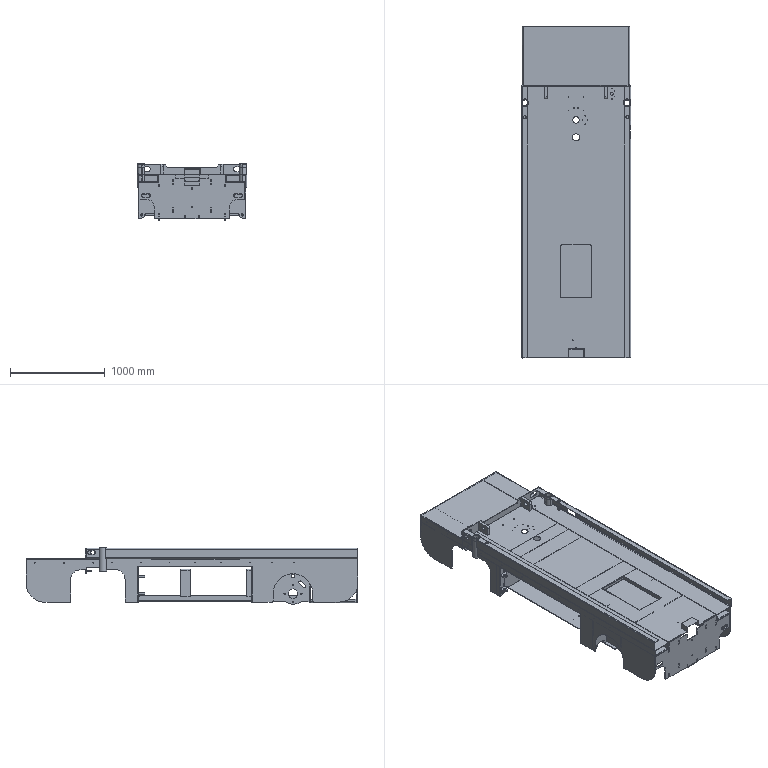Assembly | SolidWorks | mm | 35 component files | 35 solids | 1485 faces | box 1159 x 3506 x 598.09 mm | volume 81128529 mm3 | plane 1002 | cylinder 456 | cone 16 | spline 11 | commonest cylinder face diameters 7.2 x48 10 x40 20 x27 5.2 x24 8 x18 40 x17 30 x16 13.1 x16
Bill of materials:
BodyMainBoard | 1 | Q235 | Long rectangular plate formed from thin sheet, with a shallow flange bent up along each long edge (a shallow channel). It has a large rectangular cutout, several round holes near one end, and small tabs with holes at that end.
BodySidePlate,Right | 1 | Q235 | Long, narrow, thin profiled plate/bracket. One long edge is straight; the other has two downward legs and a large semicircular arch cutout between them. A narrow bent lip runs along part of the top edge.
BoxSupport,Left | 1 | Q235 | Long L-section angle formed from sheet, with one wide leg and one short upturned flange. The short flange has notches along its length, and one end has stepped notches.
BoxSupport,Right | 1 | Q235 | Long L-section angle formed from sheet, with notches along the short flange and a stepped notch profile at one end of the wide leg. It appears to be the opposite-hand version of a similar angle part.
BrakeMountingPlate | 2 | Q235 | Flat, roughly rectangular plate with small rectangular tabs on its side edges and a rounded lobe extending from the bottom edge. It has a large central round hole surrounded by four small holes, plus a separate round hole and a diagonal slot.
CounterweightFixingFrame | 2 | Q235 | U-shaped strap or bracket formed from thin sheet: a flat top web with two long parallel legs, and a single round hole in the center of the web.
ForkliftBasePlate | 2 | Q235 | Plain straight U-channel formed from sheet: a flat base with two parallel side walls of equal height and no visible holes.
ForkliftSidePlate,Left | 1 | Q235 | Long, slender L-section angle formed from sheet. It has a semicircular edge notch near one end, a hole in the upright flange, and several small slits or marks along the flat leg.
ForkliftSidePlate,Right | 1 | Q235 | Long, slender L-section angle, apparently the opposite-hand version of a similar part. It has a semicircular edge notch near one end, an obround hole in the flange, and small slits along the flat leg.
ForkLug | 2 | Q235 | Small, thick rectangular block or plate with one large rounded corner, one smaller rounded corner, and a single round through-hole.
FrontEndPlate,2 | 1 | Q235 | Flat, elongated thin plate with a straight top edge and a profiled bottom edge with chamfered steps. It has one centered obround slot near the bottom edge.
FrontEndPlate | 1 | Q235 | Flat, elongated thin plate with obround slots near both ends, a recessed or stepped profile along the top edge, and chamfered lower corners. Two small rectangular slots are near the center.
FrontGuard | 1 | Q235 | Thin-wall cover shaped like an inverted U: a flat rectangular top panel with two matching side panels bent down. Each side panel has a stepped tab at one end, a notch with a rounded inside corner, and a large-radius rounded corner at the other end.
FrontStiffener,Left | 1 | Q235 | Long thin L-shaped angle profile: a wide flat leg and a shorter upright leg joined by a rounded bend. One corner of the flat leg has a small chamfer.
FrontStiffener,Right | 1 | Q235 | Long thin L-shaped angle profile that looks like a mirror image of the similar angle part: a wide flat leg and an upright leg on the opposite side, joined by a rounded bend, with a small chamfer on one corner of the flat leg.
FrontUprightPlate | 1 | Q235 | Flat thin plate, roughly rectangular, with a raised centre section along the top edge, stepped edges, and many through-features: two vertical obround slots, several rectangular slots, small round holes, and rounded corner lugs with round holes at the two bottom corners.
LadderFixingPlate | 1 | Q235 | Flat thin plate with a stepped, castellated top edge and wide side wings. Each wing has a horizontal obround slot and a large-radius curved cut where it meets the narrower lower body. The plate has several narrow vertical rectangular slots and two small round holes on the centreline.
MainBoardLowerBucklePlate | 1 | Q235 | Shallow open rectangular tray: a flat rectangular base with short upright walls on all four sides.
ManualPumpProtectionBox | 1 | Q235 | Inverted U-shaped channel or cover: a flat rectangular top panel with two parallel side walls bent down at rounded bends, and small circular relief notches at the ends of the bends.
RearUprightPlate | 2 | Q235 | Flat thin plate, roughly rectangular, with a tall narrow tab rising at one upper corner, a small tab on the top edge, a rectangular slot near the top-left, two notches in the bottom edge, and a rounded lug with a round hole at the lower-right corner.
RearUprightPlateConnection | 1 | Q235 | Flat thin plate with a stepped top edge (two raised blocks with a recessed centre), wide side wings joined to a narrower lower body by large concave radii, narrow vertical rectangular slots near the corners, and small notches in the top and bottom edges. No obround slots or round holes are visible.
SteeringLug | 1 | Q235 | Small thick flat plate or bracket shaped roughly like a tapered trapezoid: one angled edge, a rectangular tab on the top edge, a rounded bottom end, and one large round through-hole near the rounded end.
Stiffener,RearConnection | 1 | Q235 | Long U-shaped channel: a flat base with two parallel upright side walls joined by rounded bends, with a constant cross-section along the length.
VehicleBodyLowerLug | 2 | Q235 | Small thick flat plate or bracket with a stepped top edge (two levels of rectangular steps), one straight side, an angled lower edge, a rounded bottom end, and one large round through-hole near the rounded end.
VehicleBodySidePlate,Left | 1 | Q235 | Long, thin, flat plate with a straight top edge. The left end has a large semicircular cutout open to the bottom edge and one rounded bottom corner. A long rectangular opening runs between two narrow vertical legs. Each leg has a short bent tab with small holes and a rounded end with a single larger hole. The right end has a concave radiused notch.
VehicleBodyUpperLug | 2 | Q235 | Flat plate of even thickness with a stepped, tapering outline. It has one round through-hole near a rounded lobe at one end. Opposite the hole, one edge is stepped like a staircase, and a long straight edge slants back toward the lobe.
VerticalShaftSleeve | 2 | Q235 | Straight hollow cylindrical tube with a thin wall and plain ends. It has one small radial hole through the wall, partway along its length.
Mates:
1. coincident | BodyMainBoard-1 face at (-1392.449, -1040.568, 2815.705) dir (0, 0, -1) | ForkliftSidePlate,Right-1 face at (-1178.654, 634.006, 2815.705) dir (0, 0, 1)
2. concentric | BodyMainBoard-1 face at (-1356.654, 1601.474, 2820.705) dir (0, 0, 1) r 40.25 | ForkliftSidePlate,Right-1 face at (-1356.654, 1601.474, 2740.705) dir (0, 0, 1) r 40.25
3. parallel | BodyMainBoard-1 face at (-1392.654, -1040.568, 2823.29) dir (-1, 0, 0) | ForkliftSidePlate,Right-1 face at (-1377.654, 634.006, 2740.705) dir (-1, 0, 0)
4. coincident | BodyMainBoard-1 face at (-1392.449, -1040.568, 2815.705) dir (0, 0, -1) | ForkliftSidePlate,Left-1 face at (-455.654, 634.006, 2815.705) dir (0, 0, 1)
5. concentric | BodyMainBoard-1 face at (-277.654, 1601.474, 2820.705) dir (0, 0, 1) r 40.25 | ForkliftSidePlate,Left-1 face at (-277.654, 1601.474, 2740.705) dir (0, 0, 1) r 40.25
6. coincident | ForkliftSidePlate,Right-1 face at (-1377.654, 634.006, 2740.705) dir (-1, 0, 0) | VehicleBodySidePlate,Left-1 face at (-1377.654, 1009.2, 2306.758) dir (1, 0, 0)
7. coincident | ForkliftSidePlate,Left-1 face at (-256.654, 634.006, 2740.705) dir (1, 0, 0) | BodySidePlate,Right-1 face at (-256.654, 1009.2, 2306.758) dir (-1, 0, 0)
8. coincident | BodyMainBoard-1 face at (-1392.449, -1040.568, 2815.705) dir (0, 0, -1) | BodySidePlate,Right-1 face at (-256.654, 1009.2, 2815.705) dir (0, 0, 1)
9. coincident | ForkliftSidePlate,Right-1 face at (-458.055, 634.006, 2735.705) dir (0, 0, -1) | FrontUprightPlate-1 face at (-2022.148, 1276.474, 2735.705) dir (0, 0, 1)
10. coincident | ForkliftSidePlate,Right-1 face at (-1343.154, 634.006, 2740.705) dir (1, 0, 0) | FrontUprightPlate-1 face at (-1343.154, 1276.474, 2221.675) dir (-1, 0, 0)
11. coincident | ForkliftSidePlate,Right-1 face at (-458.055, 1286.474, 2740.705) dir (0, -1, 0) | FrontUprightPlate-1 face at (-2022.148, 1286.474, 2221.675) dir (0, 1, 0)
12. coincident | ForkliftSidePlate,Left-1 face at (-1176.253, -155.326, 2740.705) dir (0, -1, 0) | RearUprightPlate-1 face at (3301.77, -155.326, 514.924) dir (0, 1, 0)
13. coincident | ForkliftSidePlate,Left-1 face at (-331.154, 634.006, 2740.705) dir (1, 0, 0) | RearUprightPlate-1 face at (-331.154, -155.326, 514.924) dir (-1, 0, 0)
14. coincident | ForkliftSidePlate,Right-1 face at (-458.055, -155.326, 2740.705) dir (0, -1, 0) | RearUprightPlate-2 face at (-4936.078, -155.326, 514.924) dir (0, 1, 0)
15. coincident | RearUprightPlate-1 face at (3301.77, -155.326, 2397.705) dir (0, 0, -1) | BrakeMountingPlate-1 face at (-470.054, -14.958, 2397.705) dir (0, 0, 1)
16. coincident | RearUprightPlate-1 face at (-460.054, -155.326, 514.924) dir (-1, 0, 0) | BrakeMountingPlate-1 face at (-460.054, -14.958, 2306.634) dir (1, 0, 0)
17. coincident | RearUprightPlate-1 face at (3301.77, -165.326, 514.924) dir (0, -1, 0) | BrakeMountingPlate-1 face at (-470.054, -165.326, 2306.634) dir (0, 1, 0)
18. coincident | RearUprightPlate-2 face at (-1174.254, -165.326, 514.924) dir (1, 0, 0) | BrakeMountingPlate-2 face at (-1174.254, -14.958, 2306.634) dir (-1, 0, 0)
19. coincident | RearUprightPlate-2 face at (-4936.078, -165.326, 514.924) dir (0, -1, 0) | BrakeMountingPlate-2 face at (-1174.254, -165.326, 2306.634) dir (0, 1, 0)
20. coincident | RearUprightPlate-2 face at (-4936.078, -165.326, 2397.705) dir (0, 0, -1) | BrakeMountingPlate-2 face at (-1174.254, -14.958, 2397.705) dir (0, 0, 1)
21. concentric | BodyMainBoard-1 face at (-1356.654, 1601.474, 2820.705) dir (0, 0, 1) r 40.25 | VerticalShaftSleeve-1 face at (-1356.654, 1601.474, 2678.295) dir (0, 0, 1) r 40
22. distance | VerticalShaftSleeve-1 face at (-1356.654, 1601.474, 2931.295) dir (0, 0, 1) | BodyMainBoard-1 face at (-1487.869, -1040.568, 2926.295) dir (0, 0, 1)
23. distance | VerticalShaftSleeve-2 face at (-277.654, 1601.474, 2931.295) dir (0, 0, 1) | BodyMainBoard-1 face at (1006.151, -1040.568, 2926.295) dir (0, 0, 1)
24. coincident | FrontUprightPlate-1 face at (-1307.654, 1276.474, 2221.675) dir (-1, 0, 0) | VehicleBodyLowerLug-1 face at (-1307.654, 1144.825, 2439.705) dir (1, 0, 0)
25. coincident | FrontUprightPlate-1 face at (-2022.148, 1276.474, 2439.705) dir (0, 0, 1) | VehicleBodyLowerLug-1 face at (-1381.214, 1144.825, 2439.705) dir (0, 0, -1)
26. coincident | FrontUprightPlate-1 face at (-2022.148, 1286.474, 2221.675) dir (0, 1, 0) | VehicleBodyLowerLug-1 face at (-1381.214, 1286.474, 2439.705) dir (0, 1, 0)
27. coincident | FrontUprightPlate-1 face at (-2022.148, 1276.474, 2439.721) dir (0, 0, 1) | VehicleBodyLowerLug-2 face at (-253.037, 1144.825, 2439.721) dir (0, 0, -1)
28. coincident | FrontUprightPlate-1 face at (-2022.148, 1286.474, 2221.675) dir (0, 1, 0) | VehicleBodyLowerLug-2 face at (-253.037, 1286.474, 2455.721) dir (0, 1, 0)
29. coincident | FrontUprightPlate-1 face at (-326.597, 1276.474, 2221.675) dir (1, 0, 0) | VehicleBodyLowerLug-2 edge at (-326.597, 1286.474, 2455.721) dir (0, 0, -1)
30. coincident | FrontUprightPlate-1 face at (-2022.148, 1276.474, 2619.521) dir (0, 0, 1) | VehicleBodyUpperLug-1 face at (-1424.9, 1092.251, 2619.521) dir (0, 0, -1)
31. coincident | FrontUprightPlate-1 face at (-2022.148, 1286.474, 2221.675) dir (0, 1, 0) | VehicleBodyUpperLug-1 face at (-1424.9, 1286.474, 2619.521) dir (0, 1, 0)
32. coincident | FrontUprightPlate-1 face at (-1257.654, 1276.474, 2221.675) dir (-1, 0, 0) | VehicleBodyUpperLug-1 face at (-1257.654, 1092.251, 2619.521) dir (1, 0, 0)
33. coincident | BrakeMountingPlate-1 face at (-470.054, -577.326, 2306.634) dir (0, -1, 0) | RearUprightPlateConnection-1 face at (-1412.879, -577.326, 2272.431) dir (0, 1, 0)
34. coincident | BrakeMountingPlate-1 face at (-470.054, -14.958, 2306.634) dir (-1, 0, 0) | RearUprightPlateConnection-1 face at (-470.054, -587.326, 2272.431) dir (1, 0, 0)
35. coincident | BodySidePlate,Right-1 face at (-475.431, 1226.474, 2306.758) dir (0, -1, 0) | VehicleBodyLowerLug-2 face at (-253.037, 1226.474, 2455.721) dir (0, 1, 0)
36. coincident | BodyMainBoard-1 face at (-1392.449, -1040.568, 2815.705) dir (0, 0, -1) | VehicleBodySidePlate,Left-1 face at (-1377.654, 1009.2, 2815.705) dir (0, 0, 1)
37. coincident | VehicleBodySidePlate,Left-1 face at (-1158.878, 1226.474, 2306.758) dir (0, -1, 0) | VehicleBodyUpperLug-1 face at (-1424.9, 1226.474, 2619.521) dir (0, 1, 0)
38. coincident | BodyMainBoard-1 face at (-1392.449, 1777.474, 2820.705) dir (0, 1, 0) | FrontEndPlate-1 face at (-1385.335, 1777.474, 2333.763) dir (0, -1, 0)
39. coincident | BodyMainBoard-1 face at (-240.654, -1040.568, 1671.7) dir (1, 0, 0) | FrontEndPlate-1 face at (-240.654, 1777.474, 2333.763) dir (1, 0, 0)
40. coincident | BodyMainBoard-1 face at (-1487.869, -1040.568, 2926.295) dir (0, 0, 1) | FrontEndPlate-1 face at (-1385.335, 1777.474, 2926.295) dir (0, 0, 1)
41. concentric | BodyMainBoard-1 face at (-277.654, 1601.474, 2820.705) dir (0, 0, 1) r 40.25 | VerticalShaftSleeve-2 face at (-277.654, 1601.474, 2678.295) dir (0, 0, 1) r 30.1
42. distance | FrontGuard-1 face at (-256.154, 1942.416, 4528.778) dir (-1, 0, 0) | ForkliftSidePlate,Left-1 face at (-256.654, 634.006, 2740.705) dir (1, 0, 0)
43. coincident | BodyMainBoard-1 face at (-1392.449, -1040.568, 2815.705) dir (0, 0, -1) | FrontGuard-1 face at (-1971.587, 1942.416, 2815.705) dir (0, 0, 1)
44. coincident | FrontEndPlate-1 face at (-1385.335, 1787.474, 2333.763) dir (0, 1, 0) | FrontGuard-1 face at (-1971.587, 1787.474, 2810.705) dir (0, -1, 0)
45. coincident | FrontGuard-1 face at (-1378.154, 1942.416, 2219.912) dir (1, 0, 0) | FrontStiffener,Left-1 face at (-1378.154, 2382.474, 2733.928) dir (-1, 0, 0)
46. coincident | FrontEndPlate-1 face at (-1385.335, 1787.474, 2333.763) dir (0, 1, 0) | FrontStiffener,Left-1 face at (-1176.514, 1787.474, 2806.289) dir (0, -1, 0)
47. coincident | FrontGuard-1 face at (-256.154, 1942.416, 4528.778) dir (-1, 0, 0) | FrontStiffener,Right-1 face at (-256.154, 2382.474, 2738.345) dir (1, 0, 0)
48. coincident | FrontGuard-1 face at (-1971.587, 1942.416, 2810.705) dir (0, 0, -1) | FrontStiffener,Right-1 face at (-457.794, 2402.474, 2810.705) dir (0, 0, 1)
49. coincident | FrontEndPlate-1 face at (-1385.335, 1787.474, 2333.763) dir (0, 1, 0) | FrontStiffener,Right-1 face at (-532.794, 1787.474, 2738.345) dir (0, -1, 0)
50. coincident | FrontStiffener,Right-1 face at (-532.794, 2402.474, 2738.345) dir (0, 1, 0) | FrontEndPlate,2-1 face at (-759.311, 2402.474, 2748.087) dir (0, -1, 0)
51. coincident | FrontGuard-1 face at (-256.154, 1942.416, 4528.778) dir (-1, 0, 0) | FrontEndPlate,2-1 face at (-256.154, 2412.474, 2748.087) dir (1, 0, 0)
52. coincident | FrontGuard-1 face at (-1971.587, 1942.416, 2810.705) dir (0, 0, -1) | FrontEndPlate,2-1 face at (-759.311, 2412.474, 2810.705) dir (0, 0, 1)
53. coincident | BodyMainBoard-1 face at (-1392.449, -1040.568, 2815.705) dir (0, 0, -1) | ForkliftBasePlate-1 face at (-460.654, 926.474, 2815.705) dir (0, 0, 1)
54. coincident | ForkliftSidePlate,Left-1 face at (-460.654, 634.006, 3459.094) dir (-1, 0, 0) | ForkliftBasePlate-1 face at (-460.654, 926.474, 2740.705) dir (1, 0, 0)
55. distance | ForkliftBasePlate-1 face at (-816.904, 1126.474, 2740.705) dir (0, 1, 0) | FrontUprightPlate-1 face at (-2022.148, 1276.474, 2221.675) dir (0, -1, 0)
56. coincident | BodyMainBoard-1 face at (-1392.449, -1040.568, 2815.705) dir (0, 0, -1) | ForkliftBasePlate-2 face at (-1173.154, 306.912, 2815.705) dir (0, 0, 1)
57. coincident | ForkliftSidePlate,Left-1 face at (-460.654, 634.006, 3459.094) dir (-1, 0, 0) | ForkliftBasePlate-2 face at (-460.654, 106.912, 2740.705) dir (1, 0, 0)
58. distance | ForkliftBasePlate-2 face at (-816.904, 106.912, 2740.705) dir (0, -1, 0) | BodyMainBoard-1 edge at (-966.654, 101.912, 2815.705) dir (1, 0, 0)
59. coincident | BodyMainBoard-1 face at (-1392.449, -1040.568, 2820.705) dir (0, 0, 1) | ForkLug-1 face at (-1116.164, 1757.474, 2820.705) dir (0, 0, -1)
60. coincident | FrontEndPlate-1 face at (-1385.335, 1777.474, 2333.763) dir (0, -1, 0) | ForkLug-1 face at (-1116.164, 1777.474, 2925.705) dir (0, 1, 0)
61. coincident | BodyMainBoard-1 face at (-1392.449, -1040.568, 2820.705) dir (0, 0, 1) | ForkLug-2 face at (-486.164, 1757.474, 2820.705) dir (0, 0, -1)
62. coincident | FrontEndPlate-1 face at (-1385.335, 1777.474, 2333.763) dir (0, -1, 0) | ForkLug-2 face at (-486.164, 1777.474, 2925.705) dir (0, 1, 0)
63. distance | ForkLug-1 face at (-1116.164, 1767.474, 2830.705) dir (1, 0, 0) | ForkLug-2 face at (-516.164, 1767.474, 2830.705) dir (-1, 0, 0)
64. distance | BodyMainBoard-1 face at (-1328.364, -1040.568, 2921.295) dir (1, 0, 0) | ForkLug-1 face at (-1146.164, 1767.474, 2830.705) dir (-1, 0, 0)
65. distance | LadderFixingPlate-1 face at (-979.858, -1083.526, 2598.898) dir (0, -1, 0) | ForkliftSidePlate,Right-1 face at (-1178.654, -1093.526, 3459.094) dir (0, -1, 0)
66. coincident | VehicleBodySidePlate,Left-1 face at (-1377.654, 1009.2, 2306.758) dir (1, 0, 0) | LadderFixingPlate-1 face at (-1377.654, -1083.526, 2598.898) dir (-1, 0, 0)
67. coincident | FrontUprightPlate-1 face at (-2022.148, 1276.474, 2619.537) dir (0, 0, 1) | VehicleBodyUpperLug-2 face at (-209.351, 1092.251, 2619.537) dir (0, 0, -1)
68. coincident | FrontUprightPlate-1 face at (-376.597, 1276.474, 2221.675) dir (1, 0, 0) | VehicleBodyUpperLug-2 face at (-376.597, 1092.251, 2635.537) dir (-1, 0, 0)
69. coincident | LadderFixingPlate-1 face at (-892.654, -1083.526, 2598.898) dir (1, 0, 0) | Stiffener,RearConnection-1 face at (-892.654, -830.526, 2357.705) dir (-1, 0, 0)
70. coincident | LadderFixingPlate-1 face at (-979.858, -1083.526, 2598.898) dir (0, -1, 0) | Stiffener,RearConnection-1 face at (-742.654, -1083.526, 2387.705) dir (0, -1, 0)
71. coincident | LadderFixingPlate-1 face at (-979.858, -1083.526, 2357.705) dir (0, 0, -1) | Stiffener,RearConnection-1 face at (-817.654, -830.526, 2357.705) dir (0, 0, 1)
72. coincident | FrontUprightPlate-1 face at (-975.157, 1276.474, 2221.675) dir (-1, 0, 0) | BoxSupport,Left-1 face at (-975.157, 988.75, 2156.778) dir (1, 0, 0)
73. coincident | FrontUprightPlate-1 face at (-659.094, 1276.474, 2221.675) dir (1, 0, 0) | BoxSupport,Right-2 face at (-659.094, 988.75, 2156.778) dir (-1, 0, 0)
74. coincident | BoxSupport,Left-1 face at (-983.157, 988.75, 2418.707) dir (0, 0, 1) | CounterweightFixingFrame-1 face at (-983.157, 779.475, 2418.707) dir (0, 0, -1)
75. coincident | CounterweightFixingFrame-1 face at (-983.157, 729.475, 2696.707) dir (-1, 0, 0) | BoxSupport,Left-1 face at (-983.157, 988.75, 2156.778) dir (-1, 0, 0)
76. coincident | BoxSupport,Left-1 face at (-983.157, 779.475, 2156.778) dir (0, -1, 0) | CounterweightFixingFrame-1 face at (-983.157, 779.475, 2696.707) dir (0, 1, 0)
77. coincident | BoxSupport,Left-1 face at (-983.157, 988.75, 2156.778) dir (-1, 0, 0) | CounterweightFixingFrame-2 face at (-983.157, 29.475, 2696.707) dir (-1, 0, 0)
78. coincident | BoxSupport,Left-1 face at (-983.157, 988.75, 2418.707) dir (0, 0, 1) | CounterweightFixingFrame-2 face at (-983.157, 79.475, 2418.707) dir (0, 0, -1)
79. coincident | BoxSupport,Left-1 face at (-983.157, 79.475, 2156.778) dir (0, -1, 0) | CounterweightFixingFrame-2 face at (-983.157, 79.475, 2696.707) dir (0, 1, 0)
80. coincident | BodyMainBoard-1 face at (-1392.449, -1040.568, 2815.705) dir (0, 0, -1) | MainBoardLowerBucklePlate-1 face at (-975.918, 106.912, 2815.705) dir (0, 0, 1)
81. coincident | ForkliftBasePlate-2 face at (-816.904, 106.912, 2740.705) dir (0, -1, 0) | MainBoardLowerBucklePlate-1 face at (-816.654, 106.912, 2783.705) dir (0, 1, 0)
82. coincident | BodyMainBoard-1 face at (-976.654, -1040.568, 2820.705) dir (1, 0, 0) | MainBoardLowerBucklePlate-1 face at (-976.654, -176.338, 2783.705) dir (1, 0, 0)
83. coincident | BodyMainBoard-1 face at (-1392.449, -1040.568, 2820.705) dir (0, 0, 1) | ManualPumpProtectionBox-1 face at (-897.154, -998.526, 2820.705) dir (0, 0, -1)
84. coincident | BodyMainBoard-1 face at (-897.154, -1093.526, 2810.705) dir (1, 0, 0) | ManualPumpProtectionBox-1 face at (-897.154, -998.526, 3039.505) dir (1, 0, 0)
85. coincident | BodyMainBoard-1 face at (-897.154, -998.526, 2810.705) dir (0, -1, 0) | ManualPumpProtectionBox-1 face at (-733.154, -998.526, 2875.505) dir (0, -1, 0)
86. coincident | FrontEndPlate-1 face at (-1385.335, 1777.474, 2686.363) dir (0, 0, -1) | SteeringLug-1 face at (-810.4, 1729.306, 2686.363) dir (0, 0, 1)
87. coincident | FrontEndPlate-1 face at (-808.019, 1777.474, 2333.763) dir (-1, 0, 0) | SteeringLug-1 face at (-808.019, 1777.474, 2686.363) dir (1, 0, 0)
88. coincident | FrontEndPlate-1 face at (-1385.335, 1787.474, 2333.763) dir (0, 1, 0) | SteeringLug-1 face at (-808.019, 1787.474, 2686.363) dir (0, 1, 0)
89. distance | ForkliftSidePlate,Right-1 face at (-1343.154, 634.006, 2740.705) dir (1, 0, 0) | RearUprightPlate-2 face at (-1342.154, -165.326, 514.924) dir (-1, 0, 0)
90. coincident | RearUprightPlateConnection-1 face at (-1412.879, -577.326, 2272.431) dir (0, 1, 0) | BoxSupport,Left-1 face at (-972, -577.326, 2359.705) dir (0, -1, 0)
91. coincident | RearUprightPlateConnection-1 face at (-1412.879, -577.326, 2272.431) dir (0, 1, 0) | BoxSupport,Right-2 face at (-662.251, -577.326, 2359.705) dir (0, -1, 0)
92. coincident | RearUprightPlate-2 face at (-4936.078, -165.326, 2367.705) dir (0, 0, -1) | BoxSupport,Left-1 face at (-1190.376, 988.75, 2367.705) dir (0, 0, 1)
93. coincident | RearUprightPlate-1 face at (3301.77, -155.326, 2367.705) dir (0, 0, -1) | BoxSupport,Right-2 face at (-443.875, 988.75, 2367.705) dir (0, 0, 1)
94. coincident | BodyMainBoard-1 face at (-1392.449, -1040.568, 2815.705) dir (0, 0, -1) | RearUprightPlate-1 face at (3301.77, -155.326, 2815.705) dir (0, 0, 1)
95. coincident | BodyMainBoard-1 face at (-1392.449, -1040.568, 2815.705) dir (0, 0, -1) | RearUprightPlate-2 face at (-4936.078, -165.326, 2815.705) dir (0, 0, 1)
96. coincident | BodyMainBoard-1 face at (-1392.449, -1040.568, 2815.705) dir (0, 0, -1) | RearUprightPlateConnection-1 face at (-1412.879, -587.326, 2815.705) dir (0, 0, 1)
97. coincident | BodyMainBoard-1 face at (-1392.449, -1040.568, 2815.705) dir (0, 0, -1) | LadderFixingPlate-1 face at (-979.858, -1083.526, 2815.705) dir (0, 0, 1)
98. coincident | BodySidePlate,Right-1 face at (-475.431, 1226.474, 2306.758) dir (0, -1, 0) | VehicleBodyUpperLug-2 face at (-209.351, 1226.474, 2635.537) dir (0, 1, 0)